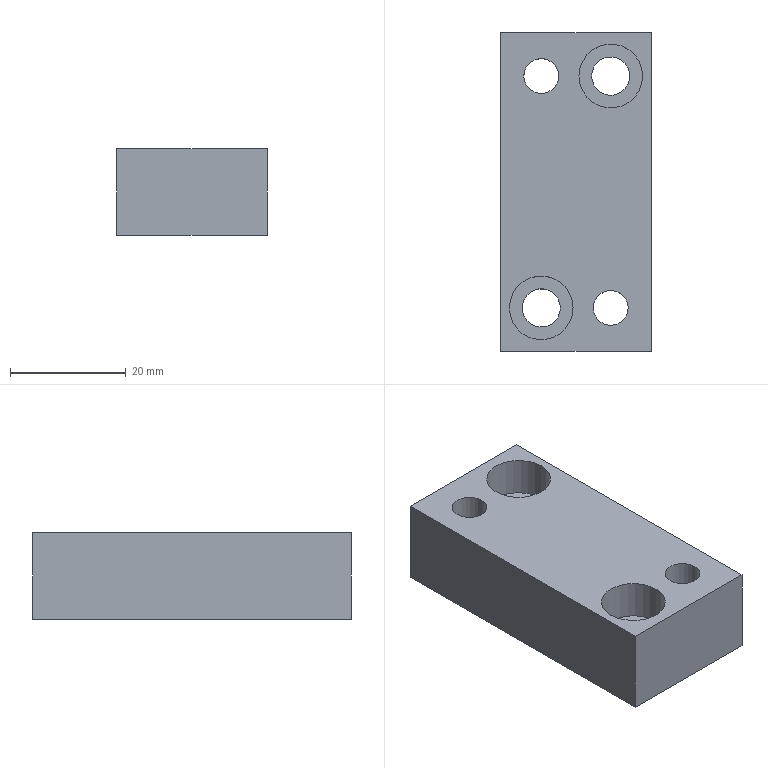Component | NX | PARALLEL_REF_BLOCK_2 | 1 solid | 14 faces | box 26 x 55 x 15 mm | volume 18748 mm3 | plane 8 | cylinder 6 | commonest cylinder face diameters 6 x2 6.6 x2 11 x2
STEP:
#1=CARTESIAN_POINT('',(0.,0.,0.));
#2=DIRECTION('',(0.,0.,1.));
#3=DIRECTION('',(1.,0.,0.));
#4=AXIS2_PLACEMENT_3D('',#1,#2,#3);
#5=CARTESIAN_POINT('',(538.625,27.591,-12.557));
#6=VERTEX_POINT('',#5);
#7=CARTESIAN_POINT('',(538.625,-27.409,-12.557));
#8=VERTEX_POINT('',#7);
#9=CARTESIAN_POINT('',(538.625,27.591,-12.557));
#10=DIRECTION('',(0.,-1.,0.));
#11=VECTOR('',#10,1.);
#12=LINE('',#9,#11);
#13=CARTESIAN_POINT('',(538.625,27.591,-27.557));
#14=DIRECTION('',(-1.,0.,0.));
#15=DIRECTION('',(0.,0.,1.));
#16=AXIS2_PLACEMENT_3D('',#13,#14,#15);
#17=PLANE('',#16);
#18=CARTESIAN_POINT('',(15.,0.));
#19=DIRECTION('',(0.,-1.));
#20=VECTOR('',#19,1.);
#21=LINE('',#18,#20);
#22=(GEOMETRIC_REPRESENTATION_CONTEXT(2)PARAMETRIC_REPRESENTATION_CONTEXT()REPRESENTATION_CONTEXT('',''));
#23=DEFINITIONAL_REPRESENTATION('',(#21),#22);
#24=PCURVE('',#17,#23);
#25=CARTESIAN_POINT('',(551.625,0.09065,-12.557));
#26=DIRECTION('',(0.,0.,1.));
#27=DIRECTION('',(1.,0.,0.));
#28=AXIS2_PLACEMENT_3D('',#25,#26,#27);
#29=PLANE('',#28);
#30=CARTESIAN_POINT('',(-13.,27.5));
#31=DIRECTION('',(0.,-1.));
#32=VECTOR('',#31,1.);
#33=LINE('',#30,#32);
#34=(GEOMETRIC_REPRESENTATION_CONTEXT(2)PARAMETRIC_REPRESENTATION_CONTEXT()REPRESENTATION_CONTEXT('',''));
#35=DEFINITIONAL_REPRESENTATION('',(#33),#34);
#36=PCURVE('',#29,#35);
#37=SURFACE_CURVE('',#12,(#24,#36),.PCURVE_S1.);
#38=EDGE_CURVE('',#6,#8,#37,.T.);
#39=ORIENTED_EDGE('',*,*,#38,.F.);
#40=CARTESIAN_POINT('',(538.625,27.591,-27.557));
#41=VERTEX_POINT('',#40);
#42=CARTESIAN_POINT('',(538.625,27.591,-27.557));
#43=DIRECTION('',(0.,0.,1.));
#44=VECTOR('',#43,1.);
#45=LINE('',#42,#44);
#46=CARTESIAN_POINT('',(0.,0.));
#47=DIRECTION('',(1.,0.));
#48=VECTOR('',#47,1.);
#49=LINE('',#46,#48);
#50=(GEOMETRIC_REPRESENTATION_CONTEXT(2)PARAMETRIC_REPRESENTATION_CONTEXT()REPRESENTATION_CONTEXT('',''));
#51=DEFINITIONAL_REPRESENTATION('',(#49),#50);
#52=PCURVE('',#17,#51);
#53=CARTESIAN_POINT('',(564.625,27.591,-27.557));
#54=DIRECTION('',(0.,1.,0.));
#55=DIRECTION('',(0.,0.,1.));
#56=AXIS2_PLACEMENT_3D('',#53,#54,#55);
#57=PLANE('',#56);
#58=CARTESIAN_POINT('',(0.,-26.));
#59=DIRECTION('',(1.,0.));
#60=VECTOR('',#59,1.);
#61=LINE('',#58,#60);
#62=(GEOMETRIC_REPRESENTATION_CONTEXT(2)PARAMETRIC_REPRESENTATION_CONTEXT()REPRESENTATION_CONTEXT('',''));
#63=DEFINITIONAL_REPRESENTATION('',(#61),#62);
#64=PCURVE('',#57,#63);
#65=SURFACE_CURVE('',#45,(#52,#64),.PCURVE_S1.);
#66=EDGE_CURVE('',#41,#6,#65,.T.);
#67=ORIENTED_EDGE('',*,*,#66,.F.);
#68=CARTESIAN_POINT('',(538.625,-27.409,-27.557));
#69=VERTEX_POINT('',#68);
#70=CARTESIAN_POINT('',(538.625,27.591,-27.557));
#71=DIRECTION('',(0.,-1.,0.));
#72=VECTOR('',#71,1.);
#73=LINE('',#70,#72);
#74=CARTESIAN_POINT('',(0.,0.));
#75=DIRECTION('',(0.,-1.));
#76=VECTOR('',#75,1.);
#77=LINE('',#74,#76);
#78=(GEOMETRIC_REPRESENTATION_CONTEXT(2)PARAMETRIC_REPRESENTATION_CONTEXT()REPRESENTATION_CONTEXT('',''));
#79=DEFINITIONAL_REPRESENTATION('',(#77),#78);
#80=PCURVE('',#17,#79);
#81=CARTESIAN_POINT('',(551.625,0.09065,-27.557));
#82=DIRECTION('',(0.,0.,1.));
#83=DIRECTION('',(1.,0.,0.));
#84=AXIS2_PLACEMENT_3D('',#81,#82,#83);
#85=PLANE('',#84);
#86=CARTESIAN_POINT('',(-13.,27.5));
#87=DIRECTION('',(0.,-1.));
#88=VECTOR('',#87,1.);
#89=LINE('',#86,#88);
#90=(GEOMETRIC_REPRESENTATION_CONTEXT(2)PARAMETRIC_REPRESENTATION_CONTEXT()REPRESENTATION_CONTEXT('',''));
#91=DEFINITIONAL_REPRESENTATION('',(#89),#90);
#92=PCURVE('',#85,#91);
#93=SURFACE_CURVE('',#73,(#80,#92),.PCURVE_S1.);
#94=EDGE_CURVE('',#41,#69,#93,.T.);
#95=ORIENTED_EDGE('',*,*,#94,.T.);
#96=CARTESIAN_POINT('',(538.625,-27.409,-27.557));
#97=DIRECTION('',(0.,0.,1.));
#98=VECTOR('',#97,1.);
#99=LINE('',#96,#98);
#100=CARTESIAN_POINT('',(0.,-55.));
#101=DIRECTION('',(1.,0.));
#102=VECTOR('',#101,1.);
#103=LINE('',#100,#102);
#104=(GEOMETRIC_REPRESENTATION_CONTEXT(2)PARAMETRIC_REPRESENTATION_CONTEXT()REPRESENTATION_CONTEXT('',''));
#105=DEFINITIONAL_REPRESENTATION('',(#103),#104);
#106=PCURVE('',#17,#105);
#107=CARTESIAN_POINT('',(538.625,-27.409,-27.557));
#108=DIRECTION('',(0.,-1.,0.));
#109=DIRECTION('',(0.,0.,-1.));
#110=AXIS2_PLACEMENT_3D('',#107,#108,#109);
#111=PLANE('',#110);
#112=CARTESIAN_POINT('',(0.,0.));
#113=DIRECTION('',(-1.,0.));
#114=VECTOR('',#113,1.);
#115=LINE('',#112,#114);
#116=(GEOMETRIC_REPRESENTATION_CONTEXT(2)PARAMETRIC_REPRESENTATION_CONTEXT()REPRESENTATION_CONTEXT('',''));
#117=DEFINITIONAL_REPRESENTATION('',(#115),#116);
#118=PCURVE('',#111,#117);
#119=SURFACE_CURVE('',#99,(#106,#118),.PCURVE_S1.);
#120=EDGE_CURVE('',#69,#8,#119,.T.);
#121=ORIENTED_EDGE('',*,*,#120,.T.);
#122=EDGE_LOOP('',(#39,#67,#95,#121));
#123=FACE_BOUND('',#122,.T.);
#124=ADVANCED_FACE('',(#123),#17,.T.);
#125=CARTESIAN_POINT('',(564.625,-27.409,-12.557));
#126=VERTEX_POINT('',#125);
#127=CARTESIAN_POINT('',(538.625,-27.409,-12.557));
#128=DIRECTION('',(1.,0.,0.));
#129=VECTOR('',#128,1.);
#130=LINE('',#127,#129);
#131=CARTESIAN_POINT('',(-15.,0.));
#132=DIRECTION('',(0.,1.));
#133=VECTOR('',#132,1.);
#134=LINE('',#131,#133);
#135=(GEOMETRIC_REPRESENTATION_CONTEXT(2)PARAMETRIC_REPRESENTATION_CONTEXT()REPRESENTATION_CONTEXT('',''));
#136=DEFINITIONAL_REPRESENTATION('',(#134),#135);
#137=PCURVE('',#111,#136);
#138=CARTESIAN_POINT('',(-13.,-27.5));
#139=DIRECTION('',(1.,0.));
#140=VECTOR('',#139,1.);
#141=LINE('',#138,#140);
#142=(GEOMETRIC_REPRESENTATION_CONTEXT(2)PARAMETRIC_REPRESENTATION_CONTEXT()REPRESENTATION_CONTEXT('',''));
#143=DEFINITIONAL_REPRESENTATION('',(#141),#142);
#144=PCURVE('',#29,#143);
#145=SURFACE_CURVE('',#130,(#137,#144),.PCURVE_S1.);
#146=EDGE_CURVE('',#8,#126,#145,.T.);
#147=ORIENTED_EDGE('',*,*,#146,.F.);
#148=ORIENTED_EDGE('',*,*,#120,.F.);
#149=CARTESIAN_POINT('',(564.625,-27.409,-27.557));
#150=VERTEX_POINT('',#149);
#151=CARTESIAN_POINT('',(538.625,-27.409,-27.557));
#152=DIRECTION('',(1.,0.,0.));
#153=VECTOR('',#152,1.);
#154=LINE('',#151,#153);
#155=CARTESIAN_POINT('',(0.,0.));
#156=DIRECTION('',(0.,1.));
#157=VECTOR('',#156,1.);
#158=LINE('',#155,#157);
#159=(GEOMETRIC_REPRESENTATION_CONTEXT(2)PARAMETRIC_REPRESENTATION_CONTEXT()REPRESENTATION_CONTEXT('',''));
#160=DEFINITIONAL_REPRESENTATION('',(#158),#159);
#161=PCURVE('',#111,#160);
#162=CARTESIAN_POINT('',(-13.,-27.5));
#163=DIRECTION('',(1.,0.));
#164=VECTOR('',#163,1.);
#165=LINE('',#162,#164);
#166=(GEOMETRIC_REPRESENTATION_CONTEXT(2)PARAMETRIC_REPRESENTATION_CONTEXT()REPRESENTATION_CONTEXT('',''));
#167=DEFINITIONAL_REPRESENTATION('',(#165),#166);
#168=PCURVE('',#85,#167);
#169=SURFACE_CURVE('',#154,(#161,#168),.PCURVE_S1.);
#170=EDGE_CURVE('',#69,#150,#169,.T.);
#171=ORIENTED_EDGE('',*,*,#170,.T.);
#172=CARTESIAN_POINT('',(564.625,-27.409,-27.557));
#173=DIRECTION('',(0.,0.,1.));
#174=VECTOR('',#173,1.);
#175=LINE('',#172,#174);
#176=CARTESIAN_POINT('',(0.,26.));
#177=DIRECTION('',(-1.,0.));
#178=VECTOR('',#177,1.);
#179=LINE('',#176,#178);
#180=(GEOMETRIC_REPRESENTATION_CONTEXT(2)PARAMETRIC_REPRESENTATION_CONTEXT()REPRESENTATION_CONTEXT('',''));
#181=DEFINITIONAL_REPRESENTATION('',(#179),#180);
#182=PCURVE('',#111,#181);
#183=CARTESIAN_POINT('',(564.625,-27.409,-27.557));
#184=DIRECTION('',(1.,0.,0.));
#185=DIRECTION('',(0.,0.,-1.));
#186=AXIS2_PLACEMENT_3D('',#183,#184,#185);
#187=PLANE('',#186);
#188=CARTESIAN_POINT('',(0.,0.));
#189=DIRECTION('',(-1.,0.));
#190=VECTOR('',#189,1.);
#191=LINE('',#188,#190);
#192=(GEOMETRIC_REPRESENTATION_CONTEXT(2)PARAMETRIC_REPRESENTATION_CONTEXT()REPRESENTATION_CONTEXT('',''));
#193=DEFINITIONAL_REPRESENTATION('',(#191),#192);
#194=PCURVE('',#187,#193);
#195=SURFACE_CURVE('',#175,(#182,#194),.PCURVE_S1.);
#196=EDGE_CURVE('',#150,#126,#195,.T.);
#197=ORIENTED_EDGE('',*,*,#196,.T.);
#198=EDGE_LOOP('',(#147,#148,#171,#197));
#199=FACE_BOUND('',#198,.T.);
#200=ADVANCED_FACE('',(#199),#111,.T.);
#201=CARTESIAN_POINT('',(564.625,27.591,-12.557));
#202=VERTEX_POINT('',#201);
#203=CARTESIAN_POINT('',(564.625,-27.409,-12.557));
#204=DIRECTION('',(0.,1.,0.));
#205=VECTOR('',#204,1.);
#206=LINE('',#203,#205);
#207=CARTESIAN_POINT('',(-15.,0.));
#208=DIRECTION('',(0.,1.));
#209=VECTOR('',#208,1.);
#210=LINE('',#207,#209);
#211=(GEOMETRIC_REPRESENTATION_CONTEXT(2)PARAMETRIC_REPRESENTATION_CONTEXT()REPRESENTATION_CONTEXT('',''));
#212=DEFINITIONAL_REPRESENTATION('',(#210),#211);
#213=PCURVE('',#187,#212);
#214=CARTESIAN_POINT('',(13.,-27.5));
#215=DIRECTION('',(0.,1.));
#216=VECTOR('',#215,1.);
#217=LINE('',#214,#216);
#218=(GEOMETRIC_REPRESENTATION_CONTEXT(2)PARAMETRIC_REPRESENTATION_CONTEXT()REPRESENTATION_CONTEXT('',''));
#219=DEFINITIONAL_REPRESENTATION('',(#217),#218);
#220=PCURVE('',#29,#219);
#221=SURFACE_CURVE('',#206,(#213,#220),.PCURVE_S1.);
#222=EDGE_CURVE('',#126,#202,#221,.T.);
#223=ORIENTED_EDGE('',*,*,#222,.F.);
#224=ORIENTED_EDGE('',*,*,#196,.F.);
#225=CARTESIAN_POINT('',(564.625,27.591,-27.557));
#226=VERTEX_POINT('',#225);
#227=CARTESIAN_POINT('',(564.625,-27.409,-27.557));
#228=DIRECTION('',(0.,1.,0.));
#229=VECTOR('',#228,1.);
#230=LINE('',#227,#229);
#231=CARTESIAN_POINT('',(0.,0.));
#232=DIRECTION('',(0.,1.));
#233=VECTOR('',#232,1.);
#234=LINE('',#231,#233);
#235=(GEOMETRIC_REPRESENTATION_CONTEXT(2)PARAMETRIC_REPRESENTATION_CONTEXT()REPRESENTATION_CONTEXT('',''));
#236=DEFINITIONAL_REPRESENTATION('',(#234),#235);
#237=PCURVE('',#187,#236);
#238=CARTESIAN_POINT('',(13.,-27.5));
#239=DIRECTION('',(0.,1.));
#240=VECTOR('',#239,1.);
#241=LINE('',#238,#240);
#242=(GEOMETRIC_REPRESENTATION_CONTEXT(2)PARAMETRIC_REPRESENTATION_CONTEXT()REPRESENTATION_CONTEXT('',''));
#243=DEFINITIONAL_REPRESENTATION('',(#241),#242);
#244=PCURVE('',#85,#243);
#245=SURFACE_CURVE('',#230,(#237,#244),.PCURVE_S1.);
#246=EDGE_CURVE('',#150,#226,#245,.T.);
#247=ORIENTED_EDGE('',*,*,#246,.T.);
#248=CARTESIAN_POINT('',(564.625,27.591,-27.557));
#249=DIRECTION('',(0.,0.,1.));
#250=VECTOR('',#249,1.);
#251=LINE('',#248,#250);
#252=CARTESIAN_POINT('',(0.,55.));
#253=DIRECTION('',(-1.,0.));
#254=VECTOR('',#253,1.);
#255=LINE('',#252,#254);
#256=(GEOMETRIC_REPRESENTATION_CONTEXT(2)PARAMETRIC_REPRESENTATION_CONTEXT()REPRESENTATION_CONTEXT('',''));
#257=DEFINITIONAL_REPRESENTATION('',(#255),#256);
#258=PCURVE('',#187,#257);
#259=CARTESIAN_POINT('',(0.,0.));
#260=DIRECTION('',(1.,0.));
#261=VECTOR('',#260,1.);
#262=LINE('',#259,#261);
#263=(GEOMETRIC_REPRESENTATION_CONTEXT(2)PARAMETRIC_REPRESENTATION_CONTEXT()REPRESENTATION_CONTEXT('',''));
#264=DEFINITIONAL_REPRESENTATION('',(#262),#263);
#265=PCURVE('',#57,#264);
#266=SURFACE_CURVE('',#251,(#258,#265),.PCURVE_S1.);
#267=EDGE_CURVE('',#226,#202,#266,.T.);
#268=ORIENTED_EDGE('',*,*,#267,.T.);
#269=EDGE_LOOP('',(#223,#224,#247,#268));
#270=FACE_BOUND('',#269,.T.);
#271=ADVANCED_FACE('',(#270),#187,.T.);
#272=CARTESIAN_POINT('',(564.625,27.591,-12.557));
#273=DIRECTION('',(-1.,0.,0.));
#274=VECTOR('',#273,1.);
#275=LINE('',#272,#274);
#276=CARTESIAN_POINT('',(15.,0.));
#277=DIRECTION('',(0.,-1.));
#278=VECTOR('',#277,1.);
#279=LINE('',#276,#278);
#280=(GEOMETRIC_REPRESENTATION_CONTEXT(2)PARAMETRIC_REPRESENTATION_CONTEXT()REPRESENTATION_CONTEXT('',''));
#281=DEFINITIONAL_REPRESENTATION('',(#279),#280);
#282=PCURVE('',#57,#281);
#283=CARTESIAN_POINT('',(13.,27.5));
#284=DIRECTION('',(-1.,0.));
#285=VECTOR('',#284,1.);
#286=LINE('',#283,#285);
#287=(GEOMETRIC_REPRESENTATION_CONTEXT(2)PARAMETRIC_REPRESENTATION_CONTEXT()REPRESENTATION_CONTEXT('',''));
#288=DEFINITIONAL_REPRESENTATION('',(#286),#287);
#289=PCURVE('',#29,#288);
#290=SURFACE_CURVE('',#275,(#282,#289),.PCURVE_S1.);
#291=EDGE_CURVE('',#202,#6,#290,.T.);
#292=ORIENTED_EDGE('',*,*,#291,.F.);
#293=ORIENTED_EDGE('',*,*,#267,.F.);
#294=CARTESIAN_POINT('',(564.625,27.591,-27.557));
#295=DIRECTION('',(-1.,0.,0.));
#296=VECTOR('',#295,1.);
#297=LINE('',#294,#296);
#298=CARTESIAN_POINT('',(0.,0.));
#299=DIRECTION('',(0.,-1.));
#300=VECTOR('',#299,1.);
#301=LINE('',#298,#300);
#302=(GEOMETRIC_REPRESENTATION_CONTEXT(2)PARAMETRIC_REPRESENTATION_CONTEXT()REPRESENTATION_CONTEXT('',''));
#303=DEFINITIONAL_REPRESENTATION('',(#301),#302);
#304=PCURVE('',#57,#303);
#305=CARTESIAN_POINT('',(13.,27.5));
#306=DIRECTION('',(-1.,0.));
#307=VECTOR('',#306,1.);
#308=LINE('',#305,#307);
#309=(GEOMETRIC_REPRESENTATION_CONTEXT(2)PARAMETRIC_REPRESENTATION_CONTEXT()REPRESENTATION_CONTEXT('',''));
#310=DEFINITIONAL_REPRESENTATION('',(#308),#309);
#311=PCURVE('',#85,#310);
#312=SURFACE_CURVE('',#297,(#304,#311),.PCURVE_S1.);
#313=EDGE_CURVE('',#226,#41,#312,.T.);
#314=ORIENTED_EDGE('',*,*,#313,.T.);
#315=ORIENTED_EDGE('',*,*,#66,.T.);
#316=EDGE_LOOP('',(#292,#293,#314,#315));
#317=FACE_BOUND('',#316,.T.);
#318=ADVANCED_FACE('',(#317),#57,.T.);
#319=CARTESIAN_POINT('',(560.925,20.091,-27.557));
#320=VERTEX_POINT('',#319);
#321=CARTESIAN_POINT('',(554.325,20.091,-27.557));
#322=VERTEX_POINT('',#321);
#323=CARTESIAN_POINT('',(557.625,20.091,-27.557));
#324=DIRECTION('',(0.,0.,1.));
#325=DIRECTION('',(1.,0.,0.));
#326=AXIS2_PLACEMENT_3D('',#323,#324,#325);
#327=CIRCLE('',#326,3.3);
#328=CARTESIAN_POINT('',(6.,20.));
#329=DIRECTION('',(1.,0.));
#330=AXIS2_PLACEMENT_2D('',#328,#329);
#331=CIRCLE('',#330,3.3);
#332=(GEOMETRIC_REPRESENTATION_CONTEXT(2)PARAMETRIC_REPRESENTATION_CONTEXT()REPRESENTATION_CONTEXT('',''));
#333=DEFINITIONAL_REPRESENTATION('',(#331),#332);
#334=PCURVE('',#85,#333);
#335=CARTESIAN_POINT('',(557.625,20.091,-47.473));
#336=DIRECTION('',(0.,0.,-1.));
#337=DIRECTION('',(-1.,0.,0.));
#338=AXIS2_PLACEMENT_3D('',#335,#336,#337);
#339=CYLINDRICAL_SURFACE('',#338,3.3);
#340=CARTESIAN_POINT('',(3.142,-19.916));
#341=DIRECTION('',(-1.,0.));
#342=VECTOR('',#341,1.);
#343=LINE('',#340,#342);
#344=(GEOMETRIC_REPRESENTATION_CONTEXT(2)PARAMETRIC_REPRESENTATION_CONTEXT()REPRESENTATION_CONTEXT('',''));
#345=DEFINITIONAL_REPRESENTATION('',(#343),#344);
#346=PCURVE('',#339,#345);
#347=SURFACE_CURVE('',#327,(#334,#346),.PCURVE_S1.);
#348=EDGE_CURVE('',#320,#322,#347,.T.);
#349=ORIENTED_EDGE('',*,*,#348,.T.);
#350=CARTESIAN_POINT('',(557.625,20.091,-27.557));
#351=DIRECTION('',(0.,0.,1.));
#352=DIRECTION('',(1.,0.,0.));
#353=AXIS2_PLACEMENT_3D('',#350,#351,#352);
#354=CIRCLE('',#353,3.3);
#355=CARTESIAN_POINT('',(6.,20.));
#356=DIRECTION('',(1.,0.));
#357=AXIS2_PLACEMENT_2D('',#355,#356);
#358=CIRCLE('',#357,3.3);
#359=(GEOMETRIC_REPRESENTATION_CONTEXT(2)PARAMETRIC_REPRESENTATION_CONTEXT()REPRESENTATION_CONTEXT('',''));
#360=DEFINITIONAL_REPRESENTATION('',(#358),#359);
#361=PCURVE('',#85,#360);
#362=CARTESIAN_POINT('',(9.425,-19.916));
#363=DIRECTION('',(-1.,0.));
#364=VECTOR('',#363,1.);
#365=LINE('',#362,#364);
#366=(GEOMETRIC_REPRESENTATION_CONTEXT(2)PARAMETRIC_REPRESENTATION_CONTEXT()REPRESENTATION_CONTEXT('',''));
#367=DEFINITIONAL_REPRESENTATION('',(#365),#366);
#368=PCURVE('',#339,#367);
#369=SURFACE_CURVE('',#354,(#361,#368),.PCURVE_S1.);
#370=EDGE_CURVE('',#322,#320,#369,.T.);
#371=ORIENTED_EDGE('',*,*,#370,.T.);
#372=EDGE_LOOP('',(#349,#371));
#373=FACE_BOUND('',#372,.T.);
#374=CARTESIAN_POINT('',(548.925,-19.909,-27.557));
#375=VERTEX_POINT('',#374);
#376=CARTESIAN_POINT('',(542.325,-19.909,-27.557));
#377=VERTEX_POINT('',#376);
#378=CARTESIAN_POINT('',(545.625,-19.909,-27.557));
#379=DIRECTION('',(0.,0.,1.));
#380=DIRECTION('',(1.,0.,0.));
#381=AXIS2_PLACEMENT_3D('',#378,#379,#380);
#382=CIRCLE('',#381,3.3);
#383=CARTESIAN_POINT('',(-6.,-20.));
#384=DIRECTION('',(1.,0.));
#385=AXIS2_PLACEMENT_2D('',#383,#384);
#386=CIRCLE('',#385,3.3);
#387=(GEOMETRIC_REPRESENTATION_CONTEXT(2)PARAMETRIC_REPRESENTATION_CONTEXT()REPRESENTATION_CONTEXT('',''));
#388=DEFINITIONAL_REPRESENTATION('',(#386),#387);
#389=PCURVE('',#85,#388);
#390=CARTESIAN_POINT('',(545.625,-19.909,-47.473));
#391=DIRECTION('',(0.,0.,-1.));
#392=DIRECTION('',(-1.,0.,0.));
#393=AXIS2_PLACEMENT_3D('',#390,#391,#392);
#394=CYLINDRICAL_SURFACE('',#393,3.3);
#395=CARTESIAN_POINT('',(3.142,-19.916));
#396=DIRECTION('',(-1.,0.));
#397=VECTOR('',#396,1.);
#398=LINE('',#395,#397);
#399=(GEOMETRIC_REPRESENTATION_CONTEXT(2)PARAMETRIC_REPRESENTATION_CONTEXT()REPRESENTATION_CONTEXT('',''));
#400=DEFINITIONAL_REPRESENTATION('',(#398),#399);
#401=PCURVE('',#394,#400);
#402=SURFACE_CURVE('',#382,(#389,#401),.PCURVE_S1.);
#403=EDGE_CURVE('',#375,#377,#402,.T.);
#404=ORIENTED_EDGE('',*,*,#403,.T.);
#405=CARTESIAN_POINT('',(545.625,-19.909,-27.557));
#406=DIRECTION('',(0.,0.,1.));
#407=DIRECTION('',(1.,0.,0.));
#408=AXIS2_PLACEMENT_3D('',#405,#406,#407);
#409=CIRCLE('',#408,3.3);
#410=CARTESIAN_POINT('',(-6.,-20.));
#411=DIRECTION('',(1.,0.));
#412=AXIS2_PLACEMENT_2D('',#410,#411);
#413=CIRCLE('',#412,3.3);
#414=(GEOMETRIC_REPRESENTATION_CONTEXT(2)PARAMETRIC_REPRESENTATION_CONTEXT()REPRESENTATION_CONTEXT('',''));
#415=DEFINITIONAL_REPRESENTATION('',(#413),#414);
#416=PCURVE('',#85,#415);
#417=CARTESIAN_POINT('',(9.425,-19.916));
#418=DIRECTION('',(-1.,0.));
#419=VECTOR('',#418,1.);
#420=LINE('',#417,#419);
#421=(GEOMETRIC_REPRESENTATION_CONTEXT(2)PARAMETRIC_REPRESENTATION_CONTEXT()REPRESENTATION_CONTEXT('',''));
#422=DEFINITIONAL_REPRESENTATION('',(#420),#421);
#423=PCURVE('',#394,#422);
#424=SURFACE_CURVE('',#409,(#416,#423),.PCURVE_S1.);
#425=EDGE_CURVE('',#377,#375,#424,.T.);
#426=ORIENTED_EDGE('',*,*,#425,.T.);
#427=EDGE_LOOP('',(#404,#426));
#428=FACE_BOUND('',#427,.T.);
#429=CARTESIAN_POINT('',(560.625,-19.909,-27.557));
#430=VERTEX_POINT('',#429);
#431=CARTESIAN_POINT('',(554.625,-19.909,-27.557));
#432=VERTEX_POINT('',#431);
#433=CARTESIAN_POINT('',(557.625,-19.909,-27.557));
#434=DIRECTION('',(0.,0.,1.));
#435=DIRECTION('',(1.,0.,0.));
#436=AXIS2_PLACEMENT_3D('',#433,#434,#435);
#437=CIRCLE('',#436,3.);
#438=CARTESIAN_POINT('',(6.,-20.));
#439=DIRECTION('',(1.,0.));
#440=AXIS2_PLACEMENT_2D('',#438,#439);
#441=CIRCLE('',#440,3.);
#442=(GEOMETRIC_REPRESENTATION_CONTEXT(2)PARAMETRIC_REPRESENTATION_CONTEXT()REPRESENTATION_CONTEXT('',''));
#443=DEFINITIONAL_REPRESENTATION('',(#441),#442);
#444=PCURVE('',#85,#443);
#445=CARTESIAN_POINT('',(557.625,-19.909,-12.557));
#446=DIRECTION('',(0.,0.,-1.));
#447=DIRECTION('',(-1.,0.,0.));
#448=AXIS2_PLACEMENT_3D('',#445,#446,#447);
#449=CYLINDRICAL_SURFACE('',#448,3.);
#450=CARTESIAN_POINT('',(3.142,15.));
#451=DIRECTION('',(-1.,0.));
#452=VECTOR('',#451,1.);
#453=LINE('',#450,#452);
#454=(GEOMETRIC_REPRESENTATION_CONTEXT(2)PARAMETRIC_REPRESENTATION_CONTEXT()REPRESENTATION_CONTEXT('',''));
#455=DEFINITIONAL_REPRESENTATION('',(#453),#454);
#456=PCURVE('',#449,#455);
#457=SURFACE_CURVE('',#437,(#444,#456),.PCURVE_S1.);
#458=EDGE_CURVE('',#430,#432,#457,.T.);
#459=ORIENTED_EDGE('',*,*,#458,.T.);
#460=CARTESIAN_POINT('',(557.625,-19.909,-27.557));
#461=DIRECTION('',(0.,0.,1.));
#462=DIRECTION('',(1.,0.,0.));
#463=AXIS2_PLACEMENT_3D('',#460,#461,#462);
#464=CIRCLE('',#463,3.);
#465=CARTESIAN_POINT('',(6.,-20.));
#466=DIRECTION('',(1.,0.));
#467=AXIS2_PLACEMENT_2D('',#465,#466);
#468=CIRCLE('',#467,3.);
#469=(GEOMETRIC_REPRESENTATION_CONTEXT(2)PARAMETRIC_REPRESENTATION_CONTEXT()REPRESENTATION_CONTEXT('',''));
#470=DEFINITIONAL_REPRESENTATION('',(#468),#469);
#471=PCURVE('',#85,#470);
#472=CARTESIAN_POINT('',(9.425,15.));
#473=DIRECTION('',(-1.,0.));
#474=VECTOR('',#473,1.);
#475=LINE('',#472,#474);
#476=(GEOMETRIC_REPRESENTATION_CONTEXT(2)PARAMETRIC_REPRESENTATION_CONTEXT()REPRESENTATION_CONTEXT('',''));
#477=DEFINITIONAL_REPRESENTATION('',(#475),#476);
#478=PCURVE('',#449,#477);
#479=SURFACE_CURVE('',#464,(#471,#478),.PCURVE_S1.);
#480=EDGE_CURVE('',#432,#430,#479,.T.);
#481=ORIENTED_EDGE('',*,*,#480,.T.);
#482=EDGE_LOOP('',(#459,#481));
#483=FACE_BOUND('',#482,.T.);
#484=CARTESIAN_POINT('',(548.625,20.091,-27.557));
#485=VERTEX_POINT('',#484);
#486=CARTESIAN_POINT('',(542.625,20.091,-27.557));
#487=VERTEX_POINT('',#486);
#488=CARTESIAN_POINT('',(545.625,20.091,-27.557));
#489=DIRECTION('',(0.,0.,1.));
#490=DIRECTION('',(1.,0.,0.));
#491=AXIS2_PLACEMENT_3D('',#488,#489,#490);
#492=CIRCLE('',#491,3.);
#493=CARTESIAN_POINT('',(-6.,20.));
#494=DIRECTION('',(1.,0.));
#495=AXIS2_PLACEMENT_2D('',#493,#494);
#496=CIRCLE('',#495,3.);
#497=(GEOMETRIC_REPRESENTATION_CONTEXT(2)PARAMETRIC_REPRESENTATION_CONTEXT()REPRESENTATION_CONTEXT('',''));
#498=DEFINITIONAL_REPRESENTATION('',(#496),#497);
#499=PCURVE('',#85,#498);
#500=CARTESIAN_POINT('',(545.625,20.091,-12.557));
#501=DIRECTION('',(0.,0.,-1.));
#502=DIRECTION('',(-1.,0.,0.));
#503=AXIS2_PLACEMENT_3D('',#500,#501,#502);
#504=CYLINDRICAL_SURFACE('',#503,3.);
#505=CARTESIAN_POINT('',(3.142,15.));
#506=DIRECTION('',(-1.,0.));
#507=VECTOR('',#506,1.);
#508=LINE('',#505,#507);
#509=(GEOMETRIC_REPRESENTATION_CONTEXT(2)PARAMETRIC_REPRESENTATION_CONTEXT()REPRESENTATION_CONTEXT('',''));
#510=DEFINITIONAL_REPRESENTATION('',(#508),#509);
#511=PCURVE('',#504,#510);
#512=SURFACE_CURVE('',#492,(#499,#511),.PCURVE_S1.);
#513=EDGE_CURVE('',#485,#487,#512,.T.);
#514=ORIENTED_EDGE('',*,*,#513,.T.);
#515=CARTESIAN_POINT('',(545.625,20.091,-27.557));
#516=DIRECTION('',(0.,0.,1.));
#517=DIRECTION('',(1.,0.,0.));
#518=AXIS2_PLACEMENT_3D('',#515,#516,#517);
#519=CIRCLE('',#518,3.);
#520=CARTESIAN_POINT('',(-6.,20.));
#521=DIRECTION('',(1.,0.));
#522=AXIS2_PLACEMENT_2D('',#520,#521);
#523=CIRCLE('',#522,3.);
#524=(GEOMETRIC_REPRESENTATION_CONTEXT(2)PARAMETRIC_REPRESENTATION_CONTEXT()REPRESENTATION_CONTEXT('',''));
#525=DEFINITIONAL_REPRESENTATION('',(#523),#524);
#526=PCURVE('',#85,#525);
#527=CARTESIAN_POINT('',(9.425,15.));
#528=DIRECTION('',(-1.,0.));
#529=VECTOR('',#528,1.);
#530=LINE('',#527,#529);
#531=(GEOMETRIC_REPRESENTATION_CONTEXT(2)PARAMETRIC_REPRESENTATION_CONTEXT()REPRESENTATION_CONTEXT('',''));
#532=DEFINITIONAL_REPRESENTATION('',(#530),#531);
#533=PCURVE('',#504,#532);
#534=SURFACE_CURVE('',#519,(#526,#533),.PCURVE_S1.);
#535=EDGE_CURVE('',#487,#485,#534,.T.);
#536=ORIENTED_EDGE('',*,*,#535,.T.);
#537=EDGE_LOOP('',(#514,#536));
#538=FACE_BOUND('',#537,.T.);
#539=ORIENTED_EDGE('',*,*,#94,.F.);
#540=ORIENTED_EDGE('',*,*,#313,.F.);
#541=ORIENTED_EDGE('',*,*,#246,.F.);
#542=ORIENTED_EDGE('',*,*,#170,.F.);
#543=EDGE_LOOP('',(#539,#540,#541,#542));
#544=FACE_BOUND('',#543,.T.);
#545=ADVANCED_FACE('',(#373,#428,#483,#538,#544),#85,.F.);
#546=CARTESIAN_POINT('',(552.125,20.091,-12.557));
#547=VERTEX_POINT('',#546);
#548=CARTESIAN_POINT('',(557.625,20.091,-12.557));
#549=DIRECTION('',(0.,0.,-1.));
#550=DIRECTION('',(-1.,0.,0.));
#551=AXIS2_PLACEMENT_3D('',#548,#549,#550);
#552=CIRCLE('',#551,5.5);
#553=CARTESIAN_POINT('',(0.5,20.));
#554=CARTESIAN_POINT('',(0.5,29.526));
#555=CARTESIAN_POINT('',(8.75,24.763));
#556=CARTESIAN_POINT('',(17.,20.));
#557=CARTESIAN_POINT('',(8.75,15.237));
#558=CARTESIAN_POINT('',(0.5,10.474));
#559=CARTESIAN_POINT('',(0.5,20.));
#560=(BOUNDED_CURVE()B_SPLINE_CURVE(2,(#553,#554,#555,#556,#557,#558,#559),.UNSPECIFIED.,.T.,.F.)B_SPLINE_CURVE_WITH_KNOTS((1,2,2,2,2,1),(-2.094,0.,2.094,4.189,6.283,8.378),.UNSPECIFIED.)CURVE()GEOMETRIC_REPRESENTATION_ITEM()RATIONAL_B_SPLINE_CURVE((1.,0.5,1.,0.5,1.,0.5,1.))REPRESENTATION_ITEM(''));
#561=(GEOMETRIC_REPRESENTATION_CONTEXT(2)PARAMETRIC_REPRESENTATION_CONTEXT()REPRESENTATION_CONTEXT('',''));
#562=DEFINITIONAL_REPRESENTATION('',(#560),#561);
#563=PCURVE('',#29,#562);
#564=CARTESIAN_POINT('',(557.625,20.091,-12.557));
#565=DIRECTION('',(0.,0.,-1.));
#566=DIRECTION('',(-1.,0.,0.));
#567=AXIS2_PLACEMENT_3D('',#564,#565,#566);
#568=CYLINDRICAL_SURFACE('',#567,5.5);
#569=CARTESIAN_POINT('',(0.,0.));
#570=DIRECTION('',(1.,0.));
#571=VECTOR('',#570,1.);
#572=LINE('',#569,#571);
#573=(GEOMETRIC_REPRESENTATION_CONTEXT(2)PARAMETRIC_REPRESENTATION_CONTEXT()REPRESENTATION_CONTEXT('',''));
#574=DEFINITIONAL_REPRESENTATION('',(#572),#573);
#575=PCURVE('',#568,#574);
#576=SURFACE_CURVE('',#552,(#563,#575),.PCURVE_S1.);
#577=EDGE_CURVE('',#547,#547,#576,.T.);
#578=ORIENTED_EDGE('',*,*,#577,.T.);
#579=EDGE_LOOP('',(#578));
#580=FACE_BOUND('',#579,.T.);
#581=CARTESIAN_POINT('',(540.125,-19.909,-12.557));
#582=VERTEX_POINT('',#581);
#583=CARTESIAN_POINT('',(545.625,-19.909,-12.557));
#584=DIRECTION('',(0.,0.,-1.));
#585=DIRECTION('',(-1.,0.,0.));
#586=AXIS2_PLACEMENT_3D('',#583,#584,#585);
#587=CIRCLE('',#586,5.5);
#588=CARTESIAN_POINT('',(-11.5,-20.));
#589=CARTESIAN_POINT('',(-11.5,-10.474));
#590=CARTESIAN_POINT('',(-3.25,-15.237));
#591=CARTESIAN_POINT('',(5.,-20.));
#592=CARTESIAN_POINT('',(-3.25,-24.763));
#593=CARTESIAN_POINT('',(-11.5,-29.526));
#594=CARTESIAN_POINT('',(-11.5,-20.));
#595=(BOUNDED_CURVE()B_SPLINE_CURVE(2,(#588,#589,#590,#591,#592,#593,#594),.UNSPECIFIED.,.T.,.F.)B_SPLINE_CURVE_WITH_KNOTS((1,2,2,2,2,1),(-2.094,0.,2.094,4.189,6.283,8.378),.UNSPECIFIED.)CURVE()GEOMETRIC_REPRESENTATION_ITEM()RATIONAL_B_SPLINE_CURVE((1.,0.5,1.,0.5,1.,0.5,1.))REPRESENTATION_ITEM(''));
#596=(GEOMETRIC_REPRESENTATION_CONTEXT(2)PARAMETRIC_REPRESENTATION_CONTEXT()REPRESENTATION_CONTEXT('',''));
#597=DEFINITIONAL_REPRESENTATION('',(#595),#596);
#598=PCURVE('',#29,#597);
#599=CARTESIAN_POINT('',(545.625,-19.909,-12.557));
#600=DIRECTION('',(0.,0.,-1.));
#601=DIRECTION('',(-1.,0.,0.));
#602=AXIS2_PLACEMENT_3D('',#599,#600,#601);
#603=CYLINDRICAL_SURFACE('',#602,5.5);
#604=CARTESIAN_POINT('',(0.,0.));
#605=DIRECTION('',(1.,0.));
#606=VECTOR('',#605,1.);
#607=LINE('',#604,#606);
#608=(GEOMETRIC_REPRESENTATION_CONTEXT(2)PARAMETRIC_REPRESENTATION_CONTEXT()REPRESENTATION_CONTEXT('',''));
#609=DEFINITIONAL_REPRESENTATION('',(#607),#608);
#610=PCURVE('',#603,#609);
#611=SURFACE_CURVE('',#587,(#598,#610),.PCURVE_S1.);
#612=EDGE_CURVE('',#582,#582,#611,.T.);
#613=ORIENTED_EDGE('',*,*,#612,.T.);
#614=EDGE_LOOP('',(#613));
#615=FACE_BOUND('',#614,.T.);
#616=CARTESIAN_POINT('',(554.625,-19.909,-12.557));
#617=VERTEX_POINT('',#616);
#618=CARTESIAN_POINT('',(557.625,-19.909,-12.557));
#619=DIRECTION('',(0.,0.,-1.));
#620=DIRECTION('',(-1.,0.,0.));
#621=AXIS2_PLACEMENT_3D('',#618,#619,#620);
#622=CIRCLE('',#621,3.);
#623=CARTESIAN_POINT('',(3.,-20.));
#624=CARTESIAN_POINT('',(3.,-14.804));
#625=CARTESIAN_POINT('',(7.5,-17.402));
#626=CARTESIAN_POINT('',(12.,-20.));
#627=CARTESIAN_POINT('',(7.5,-22.598));
#628=CARTESIAN_POINT('',(3.,-25.196));
#629=CARTESIAN_POINT('',(3.,-20.));
#630=(BOUNDED_CURVE()B_SPLINE_CURVE(2,(#623,#624,#625,#626,#627,#628,#629),.UNSPECIFIED.,.T.,.F.)B_SPLINE_CURVE_WITH_KNOTS((1,2,2,2,2,1),(-2.094,0.,2.094,4.189,6.283,8.378),.UNSPECIFIED.)CURVE()GEOMETRIC_REPRESENTATION_ITEM()RATIONAL_B_SPLINE_CURVE((1.,0.5,1.,0.5,1.,0.5,1.))REPRESENTATION_ITEM(''));
#631=(GEOMETRIC_REPRESENTATION_CONTEXT(2)PARAMETRIC_REPRESENTATION_CONTEXT()REPRESENTATION_CONTEXT('',''));
#632=DEFINITIONAL_REPRESENTATION('',(#630),#631);
#633=PCURVE('',#29,#632);
#634=CARTESIAN_POINT('',(0.,0.));
#635=DIRECTION('',(1.,0.));
#636=VECTOR('',#635,1.);
#637=LINE('',#634,#636);
#638=(GEOMETRIC_REPRESENTATION_CONTEXT(2)PARAMETRIC_REPRESENTATION_CONTEXT()REPRESENTATION_CONTEXT('',''));
#639=DEFINITIONAL_REPRESENTATION('',(#637),#638);
#640=PCURVE('',#449,#639);
#641=SURFACE_CURVE('',#622,(#633,#640),.PCURVE_S1.);
#642=EDGE_CURVE('',#617,#617,#641,.T.);
#643=ORIENTED_EDGE('',*,*,#642,.T.);
#644=EDGE_LOOP('',(#643));
#645=FACE_BOUND('',#644,.T.);
#646=CARTESIAN_POINT('',(542.625,20.091,-12.557));
#647=VERTEX_POINT('',#646);
#648=CARTESIAN_POINT('',(545.625,20.091,-12.557));
#649=DIRECTION('',(0.,0.,-1.));
#650=DIRECTION('',(-1.,0.,0.));
#651=AXIS2_PLACEMENT_3D('',#648,#649,#650);
#652=CIRCLE('',#651,3.);
#653=CARTESIAN_POINT('',(-9.,20.));
#654=CARTESIAN_POINT('',(-9.,25.196));
#655=CARTESIAN_POINT('',(-4.5,22.598));
#656=CARTESIAN_POINT('',(-0.,20.));
#657=CARTESIAN_POINT('',(-4.5,17.402));
#658=CARTESIAN_POINT('',(-9.,14.804));
#659=CARTESIAN_POINT('',(-9.,20.));
#660=(BOUNDED_CURVE()B_SPLINE_CURVE(2,(#653,#654,#655,#656,#657,#658,#659),.UNSPECIFIED.,.T.,.F.)B_SPLINE_CURVE_WITH_KNOTS((1,2,2,2,2,1),(-2.094,0.,2.094,4.189,6.283,8.378),.UNSPECIFIED.)CURVE()GEOMETRIC_REPRESENTATION_ITEM()RATIONAL_B_SPLINE_CURVE((1.,0.5,1.,0.5,1.,0.5,1.))REPRESENTATION_ITEM(''));
#661=(GEOMETRIC_REPRESENTATION_CONTEXT(2)PARAMETRIC_REPRESENTATION_CONTEXT()REPRESENTATION_CONTEXT('',''));
#662=DEFINITIONAL_REPRESENTATION('',(#660),#661);
#663=PCURVE('',#29,#662);
#664=CARTESIAN_POINT('',(0.,0.));
#665=DIRECTION('',(1.,0.));
#666=VECTOR('',#665,1.);
#667=LINE('',#664,#666);
#668=(GEOMETRIC_REPRESENTATION_CONTEXT(2)PARAMETRIC_REPRESENTATION_CONTEXT()REPRESENTATION_CONTEXT('',''));
#669=DEFINITIONAL_REPRESENTATION('',(#667),#668);
#670=PCURVE('',#504,#669);
#671=SURFACE_CURVE('',#652,(#663,#670),.PCURVE_S1.);
#672=EDGE_CURVE('',#647,#647,#671,.T.);
#673=ORIENTED_EDGE('',*,*,#672,.T.);
#674=EDGE_LOOP('',(#673));
#675=FACE_BOUND('',#674,.T.);
#676=ORIENTED_EDGE('',*,*,#38,.T.);
#677=ORIENTED_EDGE('',*,*,#146,.T.);
#678=ORIENTED_EDGE('',*,*,#222,.T.);
#679=ORIENTED_EDGE('',*,*,#291,.T.);
#680=EDGE_LOOP('',(#676,#677,#678,#679));
#681=FACE_BOUND('',#680,.T.);
#682=ADVANCED_FACE('',(#580,#615,#645,#675,#681),#29,.T.);
#683=ORIENTED_EDGE('',*,*,#672,.T.);
#684=CARTESIAN_POINT('',(542.625,20.091,-12.557));
#685=CARTESIAN_POINT('',(542.625,20.091,-27.557));
#686=B_SPLINE_CURVE_WITH_KNOTS('',1,(#684,#685),.UNSPECIFIED.,.F.,.F.,(2,2),(0.,15.),.PIECEWISE_BEZIER_KNOTS.);
#687=CARTESIAN_POINT('',(6.283,0.));
#688=DIRECTION('',(0.,1.));
#689=VECTOR('',#688,1.);
#690=LINE('',#687,#689);
#691=(GEOMETRIC_REPRESENTATION_CONTEXT(2)PARAMETRIC_REPRESENTATION_CONTEXT()REPRESENTATION_CONTEXT('',''));
#692=DEFINITIONAL_REPRESENTATION('',(#690),#691);
#693=PCURVE('',#504,#692);
#694=CARTESIAN_POINT('',(0.,0.));
#695=DIRECTION('',(0.,1.));
#696=VECTOR('',#695,1.);
#697=LINE('',#694,#696);
#698=(GEOMETRIC_REPRESENTATION_CONTEXT(2)PARAMETRIC_REPRESENTATION_CONTEXT()REPRESENTATION_CONTEXT('',''));
#699=DEFINITIONAL_REPRESENTATION('',(#697),#698);
#700=PCURVE('',#504,#699);
#701=SEAM_CURVE('',#686,(#693,#700),.PCURVE_S1.);
#702=EDGE_CURVE('',#647,#487,#701,.T.);
#703=ORIENTED_EDGE('',*,*,#702,.T.);
#704=ORIENTED_EDGE('',*,*,#535,.T.);
#705=ORIENTED_EDGE('',*,*,#513,.T.);
#706=ORIENTED_EDGE('',*,*,#702,.F.);
#707=EDGE_LOOP('',(#683,#703,#704,#705,#706));
#708=FACE_BOUND('',#707,.F.);
#709=ADVANCED_FACE('',(#708),#504,.F.);
#710=ORIENTED_EDGE('',*,*,#642,.T.);
#711=CARTESIAN_POINT('',(554.625,-19.909,-12.557));
#712=CARTESIAN_POINT('',(554.625,-19.909,-27.557));
#713=B_SPLINE_CURVE_WITH_KNOTS('',1,(#711,#712),.UNSPECIFIED.,.F.,.F.,(2,2),(0.,15.),.PIECEWISE_BEZIER_KNOTS.);
#714=CARTESIAN_POINT('',(6.283,0.));
#715=DIRECTION('',(0.,1.));
#716=VECTOR('',#715,1.);
#717=LINE('',#714,#716);
#718=(GEOMETRIC_REPRESENTATION_CONTEXT(2)PARAMETRIC_REPRESENTATION_CONTEXT()REPRESENTATION_CONTEXT('',''));
#719=DEFINITIONAL_REPRESENTATION('',(#717),#718);
#720=PCURVE('',#449,#719);
#721=CARTESIAN_POINT('',(0.,0.));
#722=DIRECTION('',(0.,1.));
#723=VECTOR('',#722,1.);
#724=LINE('',#721,#723);
#725=(GEOMETRIC_REPRESENTATION_CONTEXT(2)PARAMETRIC_REPRESENTATION_CONTEXT()REPRESENTATION_CONTEXT('',''));
#726=DEFINITIONAL_REPRESENTATION('',(#724),#725);
#727=PCURVE('',#449,#726);
#728=SEAM_CURVE('',#713,(#720,#727),.PCURVE_S1.);
#729=EDGE_CURVE('',#617,#432,#728,.T.);
#730=ORIENTED_EDGE('',*,*,#729,.T.);
#731=ORIENTED_EDGE('',*,*,#480,.T.);
#732=ORIENTED_EDGE('',*,*,#458,.T.);
#733=ORIENTED_EDGE('',*,*,#729,.F.);
#734=EDGE_LOOP('',(#710,#730,#731,#732,#733));
#735=FACE_BOUND('',#734,.F.);
#736=ADVANCED_FACE('',(#735),#449,.F.);
#737=CARTESIAN_POINT('',(542.325,-19.909,-19.357));
#738=VERTEX_POINT('',#737);
#739=CARTESIAN_POINT('',(545.625,-19.909,-19.357));
#740=DIRECTION('',(0.,0.,1.));
#741=DIRECTION('',(-1.,0.,0.));
#742=AXIS2_PLACEMENT_3D('',#739,#740,#741);
#743=CIRCLE('',#742,3.3);
#744=CARTESIAN_POINT('',(6.283,-28.116));
#745=DIRECTION('',(-1.,0.));
#746=VECTOR('',#745,1.);
#747=LINE('',#744,#746);
#748=(GEOMETRIC_REPRESENTATION_CONTEXT(2)PARAMETRIC_REPRESENTATION_CONTEXT()REPRESENTATION_CONTEXT('',''));
#749=DEFINITIONAL_REPRESENTATION('',(#747),#748);
#750=PCURVE('',#394,#749);
#751=CARTESIAN_POINT('',(545.625,-19.909,-19.357));
#752=DIRECTION('',(0.,0.,-1.));
#753=DIRECTION('',(-1.,0.,0.));
#754=AXIS2_PLACEMENT_3D('',#751,#752,#753);
#755=PLANE('',#754);
#756=CARTESIAN_POINT('',(3.3,0.));
#757=CARTESIAN_POINT('',(3.3,-5.716));
#758=CARTESIAN_POINT('',(-1.65,-2.858));
#759=CARTESIAN_POINT('',(-6.6,-0.));
#760=CARTESIAN_POINT('',(-1.65,2.858));
#761=CARTESIAN_POINT('',(3.3,5.716));
#762=CARTESIAN_POINT('',(3.3,0.));
#763=(BOUNDED_CURVE()B_SPLINE_CURVE(2,(#756,#757,#758,#759,#760,#761,#762),.UNSPECIFIED.,.T.,.F.)B_SPLINE_CURVE_WITH_KNOTS((1,2,2,2,2,1),(-2.094,0.,2.094,4.189,6.283,8.378),.UNSPECIFIED.)CURVE()GEOMETRIC_REPRESENTATION_ITEM()RATIONAL_B_SPLINE_CURVE((1.,0.5,1.,0.5,1.,0.5,1.))REPRESENTATION_ITEM(''));
#764=(GEOMETRIC_REPRESENTATION_CONTEXT(2)PARAMETRIC_REPRESENTATION_CONTEXT()REPRESENTATION_CONTEXT('',''));
#765=DEFINITIONAL_REPRESENTATION('',(#763),#764);
#766=PCURVE('',#755,#765);
#767=SURFACE_CURVE('',#743,(#750,#766),.PCURVE_S1.);
#768=EDGE_CURVE('',#738,#738,#767,.T.);
#769=ORIENTED_EDGE('',*,*,#768,.F.);
#770=CARTESIAN_POINT('',(542.325,-19.909,-19.357));
#771=CARTESIAN_POINT('',(542.325,-19.909,-27.557));
#772=B_SPLINE_CURVE_WITH_KNOTS('',1,(#770,#771),.UNSPECIFIED.,.F.,.F.,(2,2),(-28.116,-19.916),.PIECEWISE_BEZIER_KNOTS.);
#773=CARTESIAN_POINT('',(6.283,0.));
#774=DIRECTION('',(0.,1.));
#775=VECTOR('',#774,1.);
#776=LINE('',#773,#775);
#777=(GEOMETRIC_REPRESENTATION_CONTEXT(2)PARAMETRIC_REPRESENTATION_CONTEXT()REPRESENTATION_CONTEXT('',''));
#778=DEFINITIONAL_REPRESENTATION('',(#776),#777);
#779=PCURVE('',#394,#778);
#780=CARTESIAN_POINT('',(0.,0.));
#781=DIRECTION('',(0.,1.));
#782=VECTOR('',#781,1.);
#783=LINE('',#780,#782);
#784=(GEOMETRIC_REPRESENTATION_CONTEXT(2)PARAMETRIC_REPRESENTATION_CONTEXT()REPRESENTATION_CONTEXT('',''));
#785=DEFINITIONAL_REPRESENTATION('',(#783),#784);
#786=PCURVE('',#394,#785);
#787=SEAM_CURVE('',#772,(#779,#786),.PCURVE_S1.);
#788=EDGE_CURVE('',#738,#377,#787,.T.);
#789=ORIENTED_EDGE('',*,*,#788,.T.);
#790=ORIENTED_EDGE('',*,*,#425,.T.);
#791=ORIENTED_EDGE('',*,*,#403,.T.);
#792=ORIENTED_EDGE('',*,*,#788,.F.);
#793=EDGE_LOOP('',(#769,#789,#790,#791,#792));
#794=FACE_BOUND('',#793,.F.);
#795=ADVANCED_FACE('',(#794),#394,.F.);
#796=ORIENTED_EDGE('',*,*,#768,.F.);
#797=EDGE_LOOP('',(#796));
#798=FACE_BOUND('',#797,.T.);
#799=CARTESIAN_POINT('',(540.125,-19.909,-19.357));
#800=VERTEX_POINT('',#799);
#801=CARTESIAN_POINT('',(545.625,-19.909,-19.357));
#802=DIRECTION('',(0.,0.,1.));
#803=DIRECTION('',(-1.,0.,0.));
#804=AXIS2_PLACEMENT_3D('',#801,#802,#803);
#805=CIRCLE('',#804,5.5);
#806=CARTESIAN_POINT('',(5.5,0.));
#807=CARTESIAN_POINT('',(5.5,-9.526));
#808=CARTESIAN_POINT('',(-2.75,-4.763));
#809=CARTESIAN_POINT('',(-11.,-0.));
#810=CARTESIAN_POINT('',(-2.75,4.763));
#811=CARTESIAN_POINT('',(5.5,9.526));
#812=CARTESIAN_POINT('',(5.5,0.));
#813=(BOUNDED_CURVE()B_SPLINE_CURVE(2,(#806,#807,#808,#809,#810,#811,#812),.UNSPECIFIED.,.T.,.F.)B_SPLINE_CURVE_WITH_KNOTS((1,2,2,2,2,1),(-2.094,0.,2.094,4.189,6.283,8.378),.UNSPECIFIED.)CURVE()GEOMETRIC_REPRESENTATION_ITEM()RATIONAL_B_SPLINE_CURVE((1.,0.5,1.,0.5,1.,0.5,1.))REPRESENTATION_ITEM(''));
#814=(GEOMETRIC_REPRESENTATION_CONTEXT(2)PARAMETRIC_REPRESENTATION_CONTEXT()REPRESENTATION_CONTEXT('',''));
#815=DEFINITIONAL_REPRESENTATION('',(#813),#814);
#816=PCURVE('',#755,#815);
#817=CARTESIAN_POINT('',(6.283,6.8));
#818=DIRECTION('',(-1.,0.));
#819=VECTOR('',#818,1.);
#820=LINE('',#817,#819);
#821=(GEOMETRIC_REPRESENTATION_CONTEXT(2)PARAMETRIC_REPRESENTATION_CONTEXT()REPRESENTATION_CONTEXT('',''));
#822=DEFINITIONAL_REPRESENTATION('',(#820),#821);
#823=PCURVE('',#603,#822);
#824=SURFACE_CURVE('',#805,(#816,#823),.PCURVE_S1.);
#825=EDGE_CURVE('',#800,#800,#824,.T.);
#826=ORIENTED_EDGE('',*,*,#825,.T.);
#827=EDGE_LOOP('',(#826));
#828=FACE_BOUND('',#827,.T.);
#829=ADVANCED_FACE('',(#798,#828),#755,.F.);
#830=ORIENTED_EDGE('',*,*,#825,.T.);
#831=CARTESIAN_POINT('',(540.125,-19.909,-12.557));
#832=CARTESIAN_POINT('',(540.125,-19.909,-19.357));
#833=B_SPLINE_CURVE_WITH_KNOTS('',1,(#831,#832),.UNSPECIFIED.,.F.,.F.,(2,2),(0.,6.8),.PIECEWISE_BEZIER_KNOTS.);
#834=CARTESIAN_POINT('',(0.,0.));
#835=DIRECTION('',(0.,1.));
#836=VECTOR('',#835,1.);
#837=LINE('',#834,#836);
#838=(GEOMETRIC_REPRESENTATION_CONTEXT(2)PARAMETRIC_REPRESENTATION_CONTEXT()REPRESENTATION_CONTEXT('',''));
#839=DEFINITIONAL_REPRESENTATION('',(#837),#838);
#840=PCURVE('',#603,#839);
#841=CARTESIAN_POINT('',(6.283,0.));
#842=DIRECTION('',(0.,1.));
#843=VECTOR('',#842,1.);
#844=LINE('',#841,#843);
#845=(GEOMETRIC_REPRESENTATION_CONTEXT(2)PARAMETRIC_REPRESENTATION_CONTEXT()REPRESENTATION_CONTEXT('',''));
#846=DEFINITIONAL_REPRESENTATION('',(#844),#845);
#847=PCURVE('',#603,#846);
#848=SEAM_CURVE('',#833,(#840,#847),.PCURVE_S1.);
#849=EDGE_CURVE('',#582,#800,#848,.T.);
#850=ORIENTED_EDGE('',*,*,#849,.F.);
#851=ORIENTED_EDGE('',*,*,#612,.T.);
#852=ORIENTED_EDGE('',*,*,#849,.T.);
#853=EDGE_LOOP('',(#830,#850,#851,#852));
#854=FACE_BOUND('',#853,.F.);
#855=ADVANCED_FACE('',(#854),#603,.F.);
#856=CARTESIAN_POINT('',(554.325,20.091,-19.357));
#857=VERTEX_POINT('',#856);
#858=CARTESIAN_POINT('',(557.625,20.091,-19.357));
#859=DIRECTION('',(0.,0.,1.));
#860=DIRECTION('',(-1.,0.,0.));
#861=AXIS2_PLACEMENT_3D('',#858,#859,#860);
#862=CIRCLE('',#861,3.3);
#863=CARTESIAN_POINT('',(6.283,-28.116));
#864=DIRECTION('',(-1.,0.));
#865=VECTOR('',#864,1.);
#866=LINE('',#863,#865);
#867=(GEOMETRIC_REPRESENTATION_CONTEXT(2)PARAMETRIC_REPRESENTATION_CONTEXT()REPRESENTATION_CONTEXT('',''));
#868=DEFINITIONAL_REPRESENTATION('',(#866),#867);
#869=PCURVE('',#339,#868);
#870=CARTESIAN_POINT('',(557.625,20.091,-19.357));
#871=DIRECTION('',(0.,0.,-1.));
#872=DIRECTION('',(-1.,0.,0.));
#873=AXIS2_PLACEMENT_3D('',#870,#871,#872);
#874=PLANE('',#873);
#875=CARTESIAN_POINT('',(3.3,0.));
#876=CARTESIAN_POINT('',(3.3,-5.716));
#877=CARTESIAN_POINT('',(-1.65,-2.858));
#878=CARTESIAN_POINT('',(-6.6,-0.));
#879=CARTESIAN_POINT('',(-1.65,2.858));
#880=CARTESIAN_POINT('',(3.3,5.716));
#881=CARTESIAN_POINT('',(3.3,0.));
#882=(BOUNDED_CURVE()B_SPLINE_CURVE(2,(#875,#876,#877,#878,#879,#880,#881),.UNSPECIFIED.,.T.,.F.)B_SPLINE_CURVE_WITH_KNOTS((1,2,2,2,2,1),(-2.094,0.,2.094,4.189,6.283,8.378),.UNSPECIFIED.)CURVE()GEOMETRIC_REPRESENTATION_ITEM()RATIONAL_B_SPLINE_CURVE((1.,0.5,1.,0.5,1.,0.5,1.))REPRESENTATION_ITEM(''));
#883=(GEOMETRIC_REPRESENTATION_CONTEXT(2)PARAMETRIC_REPRESENTATION_CONTEXT()REPRESENTATION_CONTEXT('',''));
#884=DEFINITIONAL_REPRESENTATION('',(#882),#883);
#885=PCURVE('',#874,#884);
#886=SURFACE_CURVE('',#862,(#869,#885),.PCURVE_S1.);
#887=EDGE_CURVE('',#857,#857,#886,.T.);
#888=ORIENTED_EDGE('',*,*,#887,.F.);
#889=CARTESIAN_POINT('',(554.325,20.091,-19.357));
#890=CARTESIAN_POINT('',(554.325,20.091,-27.557));
#891=B_SPLINE_CURVE_WITH_KNOTS('',1,(#889,#890),.UNSPECIFIED.,.F.,.F.,(2,2),(-28.116,-19.916),.PIECEWISE_BEZIER_KNOTS.);
#892=CARTESIAN_POINT('',(6.283,0.));
#893=DIRECTION('',(0.,1.));
#894=VECTOR('',#893,1.);
#895=LINE('',#892,#894);
#896=(GEOMETRIC_REPRESENTATION_CONTEXT(2)PARAMETRIC_REPRESENTATION_CONTEXT()REPRESENTATION_CONTEXT('',''));
#897=DEFINITIONAL_REPRESENTATION('',(#895),#896);
#898=PCURVE('',#339,#897);
#899=CARTESIAN_POINT('',(0.,0.));
#900=DIRECTION('',(0.,1.));
#901=VECTOR('',#900,1.);
#902=LINE('',#899,#901);
#903=(GEOMETRIC_REPRESENTATION_CONTEXT(2)PARAMETRIC_REPRESENTATION_CONTEXT()REPRESENTATION_CONTEXT('',''));
#904=DEFINITIONAL_REPRESENTATION('',(#902),#903);
#905=PCURVE('',#339,#904);
#906=SEAM_CURVE('',#891,(#898,#905),.PCURVE_S1.);
#907=EDGE_CURVE('',#857,#322,#906,.T.);
#908=ORIENTED_EDGE('',*,*,#907,.T.);
#909=ORIENTED_EDGE('',*,*,#370,.T.);
#910=ORIENTED_EDGE('',*,*,#348,.T.);
#911=ORIENTED_EDGE('',*,*,#907,.F.);
#912=EDGE_LOOP('',(#888,#908,#909,#910,#911));
#913=FACE_BOUND('',#912,.F.);
#914=ADVANCED_FACE('',(#913),#339,.F.);
#915=ORIENTED_EDGE('',*,*,#887,.F.);
#916=EDGE_LOOP('',(#915));
#917=FACE_BOUND('',#916,.T.);
#918=CARTESIAN_POINT('',(552.125,20.091,-19.357));
#919=VERTEX_POINT('',#918);
#920=CARTESIAN_POINT('',(557.625,20.091,-19.357));
#921=DIRECTION('',(0.,0.,1.));
#922=DIRECTION('',(-1.,0.,0.));
#923=AXIS2_PLACEMENT_3D('',#920,#921,#922);
#924=CIRCLE('',#923,5.5);
#925=CARTESIAN_POINT('',(5.5,0.));
#926=CARTESIAN_POINT('',(5.5,-9.526));
#927=CARTESIAN_POINT('',(-2.75,-4.763));
#928=CARTESIAN_POINT('',(-11.,-0.));
#929=CARTESIAN_POINT('',(-2.75,4.763));
#930=CARTESIAN_POINT('',(5.5,9.526));
#931=CARTESIAN_POINT('',(5.5,0.));
#932=(BOUNDED_CURVE()B_SPLINE_CURVE(2,(#925,#926,#927,#928,#929,#930,#931),.UNSPECIFIED.,.T.,.F.)B_SPLINE_CURVE_WITH_KNOTS((1,2,2,2,2,1),(-2.094,0.,2.094,4.189,6.283,8.378),.UNSPECIFIED.)CURVE()GEOMETRIC_REPRESENTATION_ITEM()RATIONAL_B_SPLINE_CURVE((1.,0.5,1.,0.5,1.,0.5,1.))REPRESENTATION_ITEM(''));
#933=(GEOMETRIC_REPRESENTATION_CONTEXT(2)PARAMETRIC_REPRESENTATION_CONTEXT()REPRESENTATION_CONTEXT('',''));
#934=DEFINITIONAL_REPRESENTATION('',(#932),#933);
#935=PCURVE('',#874,#934);
#936=CARTESIAN_POINT('',(6.283,6.8));
#937=DIRECTION('',(-1.,0.));
#938=VECTOR('',#937,1.);
#939=LINE('',#936,#938);
#940=(GEOMETRIC_REPRESENTATION_CONTEXT(2)PARAMETRIC_REPRESENTATION_CONTEXT()REPRESENTATION_CONTEXT('',''));
#941=DEFINITIONAL_REPRESENTATION('',(#939),#940);
#942=PCURVE('',#568,#941);
#943=SURFACE_CURVE('',#924,(#935,#942),.PCURVE_S1.);
#944=EDGE_CURVE('',#919,#919,#943,.T.);
#945=ORIENTED_EDGE('',*,*,#944,.T.);
#946=EDGE_LOOP('',(#945));
#947=FACE_BOUND('',#946,.T.);
#948=ADVANCED_FACE('',(#917,#947),#874,.F.);
#949=ORIENTED_EDGE('',*,*,#944,.T.);
#950=CARTESIAN_POINT('',(552.125,20.091,-12.557));
#951=CARTESIAN_POINT('',(552.125,20.091,-19.357));
#952=B_SPLINE_CURVE_WITH_KNOTS('',1,(#950,#951),.UNSPECIFIED.,.F.,.F.,(2,2),(0.,6.8),.PIECEWISE_BEZIER_KNOTS.);
#953=CARTESIAN_POINT('',(0.,0.));
#954=DIRECTION('',(0.,1.));
#955=VECTOR('',#954,1.);
#956=LINE('',#953,#955);
#957=(GEOMETRIC_REPRESENTATION_CONTEXT(2)PARAMETRIC_REPRESENTATION_CONTEXT()REPRESENTATION_CONTEXT('',''));
#958=DEFINITIONAL_REPRESENTATION('',(#956),#957);
#959=PCURVE('',#568,#958);
#960=CARTESIAN_POINT('',(6.283,0.));
#961=DIRECTION('',(0.,1.));
#962=VECTOR('',#961,1.);
#963=LINE('',#960,#962);
#964=(GEOMETRIC_REPRESENTATION_CONTEXT(2)PARAMETRIC_REPRESENTATION_CONTEXT()REPRESENTATION_CONTEXT('',''));
#965=DEFINITIONAL_REPRESENTATION('',(#963),#964);
#966=PCURVE('',#568,#965);
#967=SEAM_CURVE('',#952,(#959,#966),.PCURVE_S1.);
#968=EDGE_CURVE('',#547,#919,#967,.T.);
#969=ORIENTED_EDGE('',*,*,#968,.F.);
#970=ORIENTED_EDGE('',*,*,#577,.T.);
#971=ORIENTED_EDGE('',*,*,#968,.T.);
#972=EDGE_LOOP('',(#949,#969,#970,#971));
#973=FACE_BOUND('',#972,.F.);
#974=ADVANCED_FACE('',(#973),#568,.F.);
#975=CLOSED_SHELL('',(#124,#200,#271,#318,#545,#682,#709,#736,#795,#829,#855,#914,#948,#974));
#976=MANIFOLD_SOLID_BREP('',#975);
#977=(LENGTH_UNIT()NAMED_UNIT(*)SI_UNIT(.MILLI.,.METRE.));
#978=UNCERTAINTY_MEASURE_WITH_UNIT(LENGTH_MEASURE(0.000005),#977,'','');
#979=(NAMED_UNIT(*)PLANE_ANGLE_UNIT()SI_UNIT($,.RADIAN.));
#980=(NAMED_UNIT(*)SI_UNIT($,.STERADIAN.)SOLID_ANGLE_UNIT());
#981=(GEOMETRIC_REPRESENTATION_CONTEXT(3)GLOBAL_UNCERTAINTY_ASSIGNED_CONTEXT((#978))GLOBAL_UNIT_ASSIGNED_CONTEXT((#977,#979,#980))REPRESENTATION_CONTEXT('',''));
#982=ADVANCED_BREP_SHAPE_REPRESENTATION('',(#4,#976),#981);